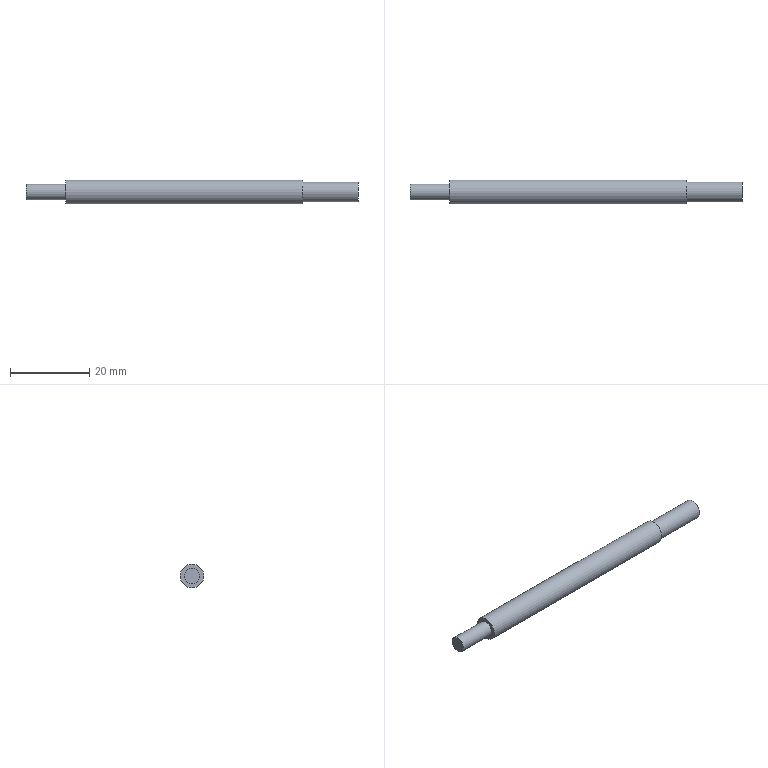Component | NX | PISTON_ROD | 1 solid | 7 faces | box 84 x 6 x 6 mm | volume 2097 mm3 | plane 4 | cylinder 3 | commonest cylinder face diameters 4 x1 6 x1 5 x1
STEP:
#1=CARTESIAN_POINT('',(0.,0.,0.));
#2=DIRECTION('',(0.,0.,1.));
#3=DIRECTION('',(1.,0.,0.));
#4=AXIS2_PLACEMENT_3D('',#1,#2,#3);
#5=CARTESIAN_POINT('',(-122.04,-20.,18.5));
#6=VERTEX_POINT('',#5);
#7=CARTESIAN_POINT('',(-122.04,-22.,18.5));
#8=DIRECTION('',(1.,0.,0.));
#9=DIRECTION('',(0.,1.,0.));
#10=AXIS2_PLACEMENT_3D('',#7,#8,#9);
#11=CIRCLE('',#10,2.);
#12=CARTESIAN_POINT('',(-122.04,-22.,18.5));
#13=DIRECTION('',(-1.,0.,0.));
#14=DIRECTION('',(0.,-1.,0.));
#15=AXIS2_PLACEMENT_3D('',#12,#13,#14);
#16=PLANE('',#15);
#17=CARTESIAN_POINT('',(-2.,0.));
#18=CARTESIAN_POINT('',(-2.,3.464));
#19=CARTESIAN_POINT('',(1.,1.732));
#20=CARTESIAN_POINT('',(4.,0.));
#21=CARTESIAN_POINT('',(1.,-1.732));
#22=CARTESIAN_POINT('',(-2.,-3.464));
#23=CARTESIAN_POINT('',(-2.,0.));
#24=(BOUNDED_CURVE()B_SPLINE_CURVE(2,(#17,#18,#19,#20,#21,#22,#23),.UNSPECIFIED.,.T.,.F.)B_SPLINE_CURVE_WITH_KNOTS((1,2,2,2,2,1),(-2.094,0.,2.094,4.189,6.283,8.378),.UNSPECIFIED.)CURVE()GEOMETRIC_REPRESENTATION_ITEM()RATIONAL_B_SPLINE_CURVE((1.,0.5,1.,0.5,1.,0.5,1.))REPRESENTATION_ITEM(''));
#25=(GEOMETRIC_REPRESENTATION_CONTEXT(2)PARAMETRIC_REPRESENTATION_CONTEXT()REPRESENTATION_CONTEXT('',''));
#26=DEFINITIONAL_REPRESENTATION('',(#24),#25);
#27=PCURVE('',#16,#26);
#28=CARTESIAN_POINT('',(-122.04,-22.,18.5));
#29=DIRECTION('',(1.,0.,0.));
#30=DIRECTION('',(0.,1.,0.));
#31=AXIS2_PLACEMENT_3D('',#28,#29,#30);
#32=CYLINDRICAL_SURFACE('',#31,2.);
#33=CARTESIAN_POINT('',(0.,0.));
#34=DIRECTION('',(1.,0.));
#35=VECTOR('',#34,1.);
#36=LINE('',#33,#35);
#37=(GEOMETRIC_REPRESENTATION_CONTEXT(2)PARAMETRIC_REPRESENTATION_CONTEXT()REPRESENTATION_CONTEXT('',''));
#38=DEFINITIONAL_REPRESENTATION('',(#36),#37);
#39=PCURVE('',#32,#38);
#40=SURFACE_CURVE('',#11,(#27,#39),.PCURVE_S1.);
#41=EDGE_CURVE('',#6,#6,#40,.T.);
#42=ORIENTED_EDGE('',*,*,#41,.F.);
#43=EDGE_LOOP('',(#42));
#44=FACE_BOUND('',#43,.T.);
#45=ADVANCED_FACE('',(#44),#16,.T.);
#46=CARTESIAN_POINT('',(-112.04,-20.,18.5));
#47=VERTEX_POINT('',#46);
#48=CARTESIAN_POINT('',(-112.04,-22.,18.5));
#49=DIRECTION('',(-1.,0.,0.));
#50=DIRECTION('',(0.,1.,0.));
#51=AXIS2_PLACEMENT_3D('',#48,#49,#50);
#52=CIRCLE('',#51,2.);
#53=CARTESIAN_POINT('',(6.283,10.));
#54=DIRECTION('',(-1.,0.));
#55=VECTOR('',#54,1.);
#56=LINE('',#53,#55);
#57=(GEOMETRIC_REPRESENTATION_CONTEXT(2)PARAMETRIC_REPRESENTATION_CONTEXT()REPRESENTATION_CONTEXT('',''));
#58=DEFINITIONAL_REPRESENTATION('',(#56),#57);
#59=PCURVE('',#32,#58);
#60=CARTESIAN_POINT('',(-112.04,-22.,18.5));
#61=DIRECTION('',(-1.,0.,0.));
#62=DIRECTION('',(0.,-1.,0.));
#63=AXIS2_PLACEMENT_3D('',#60,#61,#62);
#64=PLANE('',#63);
#65=CARTESIAN_POINT('',(0.,0.));
#66=DIRECTION('',(-1.,0.));
#67=AXIS2_PLACEMENT_2D('',#65,#66);
#68=CIRCLE('',#67,2.);
#69=(GEOMETRIC_REPRESENTATION_CONTEXT(2)PARAMETRIC_REPRESENTATION_CONTEXT()REPRESENTATION_CONTEXT('',''));
#70=DEFINITIONAL_REPRESENTATION('',(#68),#69);
#71=PCURVE('',#64,#70);
#72=SURFACE_CURVE('',#52,(#59,#71),.PCURVE_S1.);
#73=EDGE_CURVE('',#47,#47,#72,.T.);
#74=ORIENTED_EDGE('',*,*,#73,.T.);
#75=CARTESIAN_POINT('',(-122.04,-20.,18.5));
#76=CARTESIAN_POINT('',(-112.04,-20.,18.5));
#77=B_SPLINE_CURVE_WITH_KNOTS('',1,(#75,#76),.UNSPECIFIED.,.F.,.F.,(2,2),(0.,10.),.PIECEWISE_BEZIER_KNOTS.);
#78=CARTESIAN_POINT('',(0.,0.));
#79=DIRECTION('',(0.,1.));
#80=VECTOR('',#79,1.);
#81=LINE('',#78,#80);
#82=(GEOMETRIC_REPRESENTATION_CONTEXT(2)PARAMETRIC_REPRESENTATION_CONTEXT()REPRESENTATION_CONTEXT('',''));
#83=DEFINITIONAL_REPRESENTATION('',(#81),#82);
#84=PCURVE('',#32,#83);
#85=CARTESIAN_POINT('',(6.283,0.));
#86=DIRECTION('',(0.,1.));
#87=VECTOR('',#86,1.);
#88=LINE('',#85,#87);
#89=(GEOMETRIC_REPRESENTATION_CONTEXT(2)PARAMETRIC_REPRESENTATION_CONTEXT()REPRESENTATION_CONTEXT('',''));
#90=DEFINITIONAL_REPRESENTATION('',(#88),#89);
#91=PCURVE('',#32,#90);
#92=SEAM_CURVE('',#77,(#84,#91),.PCURVE_S1.);
#93=EDGE_CURVE('',#6,#47,#92,.T.);
#94=ORIENTED_EDGE('',*,*,#93,.F.);
#95=ORIENTED_EDGE('',*,*,#41,.T.);
#96=ORIENTED_EDGE('',*,*,#93,.T.);
#97=EDGE_LOOP('',(#74,#94,#95,#96));
#98=FACE_BOUND('',#97,.T.);
#99=ADVANCED_FACE('',(#98),#32,.T.);
#100=CARTESIAN_POINT('',(-52.04,-19.5,18.5));
#101=VERTEX_POINT('',#100);
#102=CARTESIAN_POINT('',(-52.04,-22.,18.5));
#103=DIRECTION('',(1.,0.,0.));
#104=DIRECTION('',(0.,1.,0.));
#105=AXIS2_PLACEMENT_3D('',#102,#103,#104);
#106=CIRCLE('',#105,2.5);
#107=CARTESIAN_POINT('',(-52.04,-22.,18.5));
#108=DIRECTION('',(1.,0.,0.));
#109=DIRECTION('',(0.,1.,0.));
#110=AXIS2_PLACEMENT_3D('',#107,#108,#109);
#111=PLANE('',#110);
#112=CARTESIAN_POINT('',(0.,0.));
#113=DIRECTION('',(1.,0.));
#114=AXIS2_PLACEMENT_2D('',#112,#113);
#115=CIRCLE('',#114,2.5);
#116=(GEOMETRIC_REPRESENTATION_CONTEXT(2)PARAMETRIC_REPRESENTATION_CONTEXT()REPRESENTATION_CONTEXT('',''));
#117=DEFINITIONAL_REPRESENTATION('',(#115),#116);
#118=PCURVE('',#111,#117);
#119=CARTESIAN_POINT('',(-52.04,-22.,18.5));
#120=DIRECTION('',(1.,0.,0.));
#121=DIRECTION('',(0.,1.,0.));
#122=AXIS2_PLACEMENT_3D('',#119,#120,#121);
#123=CYLINDRICAL_SURFACE('',#122,2.5);
#124=CARTESIAN_POINT('',(0.,0.));
#125=DIRECTION('',(1.,0.));
#126=VECTOR('',#125,1.);
#127=LINE('',#124,#126);
#128=(GEOMETRIC_REPRESENTATION_CONTEXT(2)PARAMETRIC_REPRESENTATION_CONTEXT()REPRESENTATION_CONTEXT('',''));
#129=DEFINITIONAL_REPRESENTATION('',(#127),#128);
#130=PCURVE('',#123,#129);
#131=SURFACE_CURVE('',#106,(#118,#130),.PCURVE_S1.);
#132=EDGE_CURVE('',#101,#101,#131,.T.);
#133=ORIENTED_EDGE('',*,*,#132,.F.);
#134=EDGE_LOOP('',(#133));
#135=FACE_BOUND('',#134,.T.);
#136=CARTESIAN_POINT('',(-52.04,-19.,18.5));
#137=VERTEX_POINT('',#136);
#138=CARTESIAN_POINT('',(-52.04,-22.,18.5));
#139=DIRECTION('',(1.,0.,0.));
#140=DIRECTION('',(0.,1.,0.));
#141=AXIS2_PLACEMENT_3D('',#138,#139,#140);
#142=CIRCLE('',#141,3.);
#143=CARTESIAN_POINT('',(0.,0.));
#144=DIRECTION('',(1.,0.));
#145=AXIS2_PLACEMENT_2D('',#143,#144);
#146=CIRCLE('',#145,3.);
#147=(GEOMETRIC_REPRESENTATION_CONTEXT(2)PARAMETRIC_REPRESENTATION_CONTEXT()REPRESENTATION_CONTEXT('',''));
#148=DEFINITIONAL_REPRESENTATION('',(#146),#147);
#149=PCURVE('',#111,#148);
#150=CARTESIAN_POINT('',(-112.04,-22.,18.5));
#151=DIRECTION('',(1.,0.,0.));
#152=DIRECTION('',(0.,1.,0.));
#153=AXIS2_PLACEMENT_3D('',#150,#151,#152);
#154=CYLINDRICAL_SURFACE('',#153,3.);
#155=CARTESIAN_POINT('',(0.,60.));
#156=DIRECTION('',(1.,0.));
#157=VECTOR('',#156,1.);
#158=LINE('',#155,#157);
#159=(GEOMETRIC_REPRESENTATION_CONTEXT(2)PARAMETRIC_REPRESENTATION_CONTEXT()REPRESENTATION_CONTEXT('',''));
#160=DEFINITIONAL_REPRESENTATION('',(#158),#159);
#161=PCURVE('',#154,#160);
#162=SURFACE_CURVE('',#142,(#149,#161),.PCURVE_S1.);
#163=EDGE_CURVE('',#137,#137,#162,.T.);
#164=ORIENTED_EDGE('',*,*,#163,.T.);
#165=EDGE_LOOP('',(#164));
#166=FACE_BOUND('',#165,.T.);
#167=ADVANCED_FACE('',(#135,#166),#111,.T.);
#168=ORIENTED_EDGE('',*,*,#73,.F.);
#169=EDGE_LOOP('',(#168));
#170=FACE_BOUND('',#169,.T.);
#171=CARTESIAN_POINT('',(-112.04,-19.,18.5));
#172=VERTEX_POINT('',#171);
#173=CARTESIAN_POINT('',(-112.04,-22.,18.5));
#174=DIRECTION('',(1.,0.,0.));
#175=DIRECTION('',(0.,1.,0.));
#176=AXIS2_PLACEMENT_3D('',#173,#174,#175);
#177=CIRCLE('',#176,3.);
#178=CARTESIAN_POINT('',(-3.,0.));
#179=CARTESIAN_POINT('',(-3.,5.196));
#180=CARTESIAN_POINT('',(1.5,2.598));
#181=CARTESIAN_POINT('',(6.,0.));
#182=CARTESIAN_POINT('',(1.5,-2.598));
#183=CARTESIAN_POINT('',(-3.,-5.196));
#184=CARTESIAN_POINT('',(-3.,0.));
#185=(BOUNDED_CURVE()B_SPLINE_CURVE(2,(#178,#179,#180,#181,#182,#183,#184),.UNSPECIFIED.,.T.,.F.)B_SPLINE_CURVE_WITH_KNOTS((1,2,2,2,2,1),(-2.094,0.,2.094,4.189,6.283,8.378),.UNSPECIFIED.)CURVE()GEOMETRIC_REPRESENTATION_ITEM()RATIONAL_B_SPLINE_CURVE((1.,0.5,1.,0.5,1.,0.5,1.))REPRESENTATION_ITEM(''));
#186=(GEOMETRIC_REPRESENTATION_CONTEXT(2)PARAMETRIC_REPRESENTATION_CONTEXT()REPRESENTATION_CONTEXT('',''));
#187=DEFINITIONAL_REPRESENTATION('',(#185),#186);
#188=PCURVE('',#64,#187);
#189=CARTESIAN_POINT('',(0.,0.));
#190=DIRECTION('',(1.,0.));
#191=VECTOR('',#190,1.);
#192=LINE('',#189,#191);
#193=(GEOMETRIC_REPRESENTATION_CONTEXT(2)PARAMETRIC_REPRESENTATION_CONTEXT()REPRESENTATION_CONTEXT('',''));
#194=DEFINITIONAL_REPRESENTATION('',(#192),#193);
#195=PCURVE('',#154,#194);
#196=SURFACE_CURVE('',#177,(#188,#195),.PCURVE_S1.);
#197=EDGE_CURVE('',#172,#172,#196,.T.);
#198=ORIENTED_EDGE('',*,*,#197,.F.);
#199=EDGE_LOOP('',(#198));
#200=FACE_BOUND('',#199,.T.);
#201=ADVANCED_FACE('',(#170,#200),#64,.T.);
#202=ORIENTED_EDGE('',*,*,#163,.F.);
#203=CARTESIAN_POINT('',(-112.04,-19.,18.5));
#204=CARTESIAN_POINT('',(-52.04,-19.,18.5));
#205=B_SPLINE_CURVE_WITH_KNOTS('',1,(#203,#204),.UNSPECIFIED.,.F.,.F.,(2,2),(0.,60.),.PIECEWISE_BEZIER_KNOTS.);
#206=CARTESIAN_POINT('',(0.,0.));
#207=DIRECTION('',(0.,1.));
#208=VECTOR('',#207,1.);
#209=LINE('',#206,#208);
#210=(GEOMETRIC_REPRESENTATION_CONTEXT(2)PARAMETRIC_REPRESENTATION_CONTEXT()REPRESENTATION_CONTEXT('',''));
#211=DEFINITIONAL_REPRESENTATION('',(#209),#210);
#212=PCURVE('',#154,#211);
#213=CARTESIAN_POINT('',(6.283,0.));
#214=DIRECTION('',(0.,1.));
#215=VECTOR('',#214,1.);
#216=LINE('',#213,#215);
#217=(GEOMETRIC_REPRESENTATION_CONTEXT(2)PARAMETRIC_REPRESENTATION_CONTEXT()REPRESENTATION_CONTEXT('',''));
#218=DEFINITIONAL_REPRESENTATION('',(#216),#217);
#219=PCURVE('',#154,#218);
#220=SEAM_CURVE('',#205,(#212,#219),.PCURVE_S1.);
#221=EDGE_CURVE('',#172,#137,#220,.T.);
#222=ORIENTED_EDGE('',*,*,#221,.F.);
#223=ORIENTED_EDGE('',*,*,#197,.T.);
#224=ORIENTED_EDGE('',*,*,#221,.T.);
#225=EDGE_LOOP('',(#202,#222,#223,#224));
#226=FACE_BOUND('',#225,.T.);
#227=ADVANCED_FACE('',(#226),#154,.T.);
#228=CARTESIAN_POINT('',(-38.04,-19.5,18.5));
#229=VERTEX_POINT('',#228);
#230=CARTESIAN_POINT('',(-38.04,-22.,18.5));
#231=DIRECTION('',(1.,0.,0.));
#232=DIRECTION('',(0.,1.,0.));
#233=AXIS2_PLACEMENT_3D('',#230,#231,#232);
#234=CIRCLE('',#233,2.5);
#235=CARTESIAN_POINT('',(-38.04,-22.,18.5));
#236=DIRECTION('',(1.,0.,0.));
#237=DIRECTION('',(0.,1.,0.));
#238=AXIS2_PLACEMENT_3D('',#235,#236,#237);
#239=PLANE('',#238);
#240=CARTESIAN_POINT('',(0.,0.));
#241=DIRECTION('',(1.,0.));
#242=AXIS2_PLACEMENT_2D('',#240,#241);
#243=CIRCLE('',#242,2.5);
#244=(GEOMETRIC_REPRESENTATION_CONTEXT(2)PARAMETRIC_REPRESENTATION_CONTEXT()REPRESENTATION_CONTEXT('',''));
#245=DEFINITIONAL_REPRESENTATION('',(#243),#244);
#246=PCURVE('',#239,#245);
#247=CARTESIAN_POINT('',(0.,14.));
#248=DIRECTION('',(1.,0.));
#249=VECTOR('',#248,1.);
#250=LINE('',#247,#249);
#251=(GEOMETRIC_REPRESENTATION_CONTEXT(2)PARAMETRIC_REPRESENTATION_CONTEXT()REPRESENTATION_CONTEXT('',''));
#252=DEFINITIONAL_REPRESENTATION('',(#250),#251);
#253=PCURVE('',#123,#252);
#254=SURFACE_CURVE('',#234,(#246,#253),.PCURVE_S1.);
#255=EDGE_CURVE('',#229,#229,#254,.T.);
#256=ORIENTED_EDGE('',*,*,#255,.T.);
#257=EDGE_LOOP('',(#256));
#258=FACE_BOUND('',#257,.T.);
#259=ADVANCED_FACE('',(#258),#239,.T.);
#260=ORIENTED_EDGE('',*,*,#255,.F.);
#261=CARTESIAN_POINT('',(-52.04,-19.5,18.5));
#262=CARTESIAN_POINT('',(-38.04,-19.5,18.5));
#263=B_SPLINE_CURVE_WITH_KNOTS('',1,(#261,#262),.UNSPECIFIED.,.F.,.F.,(2,2),(0.,14.),.PIECEWISE_BEZIER_KNOTS.);
#264=CARTESIAN_POINT('',(0.,0.));
#265=DIRECTION('',(0.,1.));
#266=VECTOR('',#265,1.);
#267=LINE('',#264,#266);
#268=(GEOMETRIC_REPRESENTATION_CONTEXT(2)PARAMETRIC_REPRESENTATION_CONTEXT()REPRESENTATION_CONTEXT('',''));
#269=DEFINITIONAL_REPRESENTATION('',(#267),#268);
#270=PCURVE('',#123,#269);
#271=CARTESIAN_POINT('',(6.283,0.));
#272=DIRECTION('',(0.,1.));
#273=VECTOR('',#272,1.);
#274=LINE('',#271,#273);
#275=(GEOMETRIC_REPRESENTATION_CONTEXT(2)PARAMETRIC_REPRESENTATION_CONTEXT()REPRESENTATION_CONTEXT('',''));
#276=DEFINITIONAL_REPRESENTATION('',(#274),#275);
#277=PCURVE('',#123,#276);
#278=SEAM_CURVE('',#263,(#270,#277),.PCURVE_S1.);
#279=EDGE_CURVE('',#101,#229,#278,.T.);
#280=ORIENTED_EDGE('',*,*,#279,.F.);
#281=ORIENTED_EDGE('',*,*,#132,.T.);
#282=ORIENTED_EDGE('',*,*,#279,.T.);
#283=EDGE_LOOP('',(#260,#280,#281,#282));
#284=FACE_BOUND('',#283,.T.);
#285=ADVANCED_FACE('',(#284),#123,.T.);
#286=CLOSED_SHELL('',(#45,#99,#167,#201,#227,#259,#285));
#287=MANIFOLD_SOLID_BREP('',#286);
#288=(LENGTH_UNIT()NAMED_UNIT(*)SI_UNIT(.MILLI.,.METRE.));
#289=UNCERTAINTY_MEASURE_WITH_UNIT(LENGTH_MEASURE(0.00001),#288,'','');
#290=(NAMED_UNIT(*)PLANE_ANGLE_UNIT()SI_UNIT($,.RADIAN.));
#291=(NAMED_UNIT(*)SI_UNIT($,.STERADIAN.)SOLID_ANGLE_UNIT());
#292=(GEOMETRIC_REPRESENTATION_CONTEXT(3)GLOBAL_UNCERTAINTY_ASSIGNED_CONTEXT((#289))GLOBAL_UNIT_ASSIGNED_CONTEXT((#288,#290,#291))REPRESENTATION_CONTEXT('',''));
#293=ADVANCED_BREP_SHAPE_REPRESENTATION('',(#4,#287),#292);